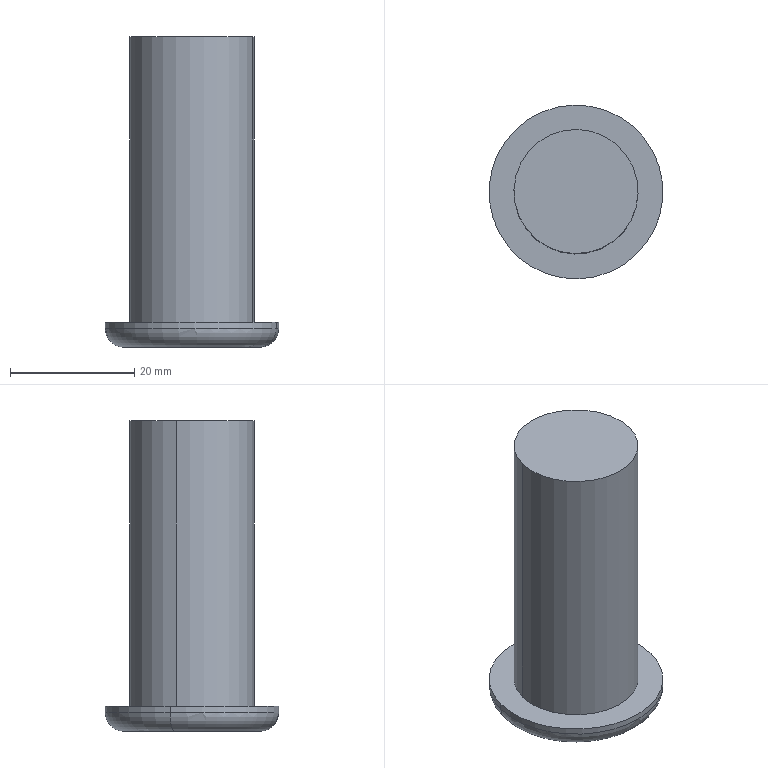Component | SolidWorks | FixedMainPin42mm-1 | 1 solid | 9 faces | box 28 x 28 x 50 mm | volume 16753 mm3 | cylinder 4 | plane 3 | torus 2 | commonest cylinder face diameters 28 x2 20 x2
build123d program:
from build123d import *

# Parameters (mm, degrees)
SKETCH1_R           = 10
BOSS_EXTRUDE1_DEPTH = 42
SKETCH2_R           = 10
BOSS_EXTRUDE2_DEPTH = 4
SKETCH3_R           = 14
BOSS_EXTRUDE3_DEPTH = 4
FILLET2_R           = 3


with BuildPart() as part:
    # Sketch1 → Boss-Extrude1 (new body)
    with BuildSketch(Plane.XY):
        with Locations(Location((0, 0, 0), (0, 0, 180))):
            Circle(SKETCH1_R)
    extrude(amount=BOSS_EXTRUDE1_DEPTH)

    # Sketch2 → Boss-Extrude2 (add)
    with BuildSketch(Plane.XY.offset(42)):
        with Locations(Location((0, 0, 0), (0, 0, 180))):
            Circle(SKETCH2_R)
    extrude(amount=BOSS_EXTRUDE2_DEPTH)

    # Sketch3 → Boss-Extrude3 (add)
    with BuildSketch(Plane.XY.offset(46)):
        Circle(SKETCH3_R)
    extrude(amount=BOSS_EXTRUDE3_DEPTH)

    # Fillet2
    fillet2_edges = [part.edges().sort_by_distance(p)[0] for p in [
        (-14, 0, 50),
    ]]
    fillet(fillet2_edges, radius=FILLET2_R)


solid = part.part

# Placed as in the assembly
solid = solid.moved(Location((17.47, 39.391, 160.846), (180, 0, 0)))
STEP:
#1=CARTESIAN_POINT('',(1.221,1.411,4.482));
#2=VERTEX_POINT('',#1);
#3=CARTESIAN_POINT('',(0.1545,1.69,4.482));
#4=VERTEX_POINT('',#3);
#5=CARTESIAN_POINT('',(0.6878,1.551,4.482));
#6=DIRECTION('',(0.,0.,1.));
#7=DIRECTION('',(-0.9675,0.2528,0.));
#8=AXIS2_PLACEMENT_3D('',#5,#6,#7);
#9=CIRCLE('',#8,0.5512);
#10=EDGE_CURVE('',#2,#4,#9,.T.);
#11=ORIENTED_EDGE('',*,*,#10,.F.);
#12=CARTESIAN_POINT('',(1.107,1.441,4.364));
#13=VERTEX_POINT('',#12);
#14=CARTESIAN_POINT('',(1.107,1.441,4.482));
#15=DIRECTION('',(0.2528,0.9675,0.));
#16=DIRECTION('',(-0.9675,0.2528,0.));
#17=AXIS2_PLACEMENT_3D('',#14,#15,#16);
#18=CIRCLE('',#17,0.1181);
#19=EDGE_CURVE('',#2,#13,#18,.T.);
#20=ORIENTED_EDGE('',*,*,#19,.T.);
#21=CARTESIAN_POINT('',(0.2688,1.66,4.364));
#22=VERTEX_POINT('',#21);
#23=CARTESIAN_POINT('',(0.6878,1.551,4.364));
#24=DIRECTION('',(0.,0.,-1.));
#25=DIRECTION('',(-0.9675,0.2528,0.));
#26=AXIS2_PLACEMENT_3D('',#23,#24,#25);
#27=CIRCLE('',#26,0.4331);
#28=EDGE_CURVE('',#22,#13,#27,.T.);
#29=ORIENTED_EDGE('',*,*,#28,.F.);
#30=CARTESIAN_POINT('',(0.2688,1.66,4.482));
#31=DIRECTION('',(-0.2528,-0.9675,0.));
#32=DIRECTION('',(0.9675,-0.2528,0.));
#33=AXIS2_PLACEMENT_3D('',#30,#31,#32);
#34=CIRCLE('',#33,0.1181);
#35=EDGE_CURVE('',#4,#22,#34,.T.);
#36=ORIENTED_EDGE('',*,*,#35,.F.);
#37=EDGE_LOOP('',(#11,#20,#29,#36));
#38=FACE_OUTER_BOUND('',#37,.T.);
#39=CARTESIAN_POINT('',(0.6878,1.551,4.482));
#40=DIRECTION('',(0.,0.,-1.));
#41=DIRECTION('',(-0.9675,0.2528,0.));
#42=AXIS2_PLACEMENT_3D('',#39,#40,#41);
#43=TOROIDAL_SURFACE('',#42,0.4331,0.1181);
#44=ADVANCED_FACE('',(#38),#43,.T.);
#45=ORIENTED_EDGE('',*,*,#10,.T.);
#46=CARTESIAN_POINT('',(0.1545,1.69,4.521));
#47=VERTEX_POINT('',#46);
#48=CARTESIAN_POINT('',(0.1545,1.69,4.364));
#49=DIRECTION('',(0.,0.,1.));
#50=VECTOR('',#49,39.37);
#51=LINE('',#48,#50);
#52=EDGE_CURVE('',#4,#47,#51,.T.);
#53=ORIENTED_EDGE('',*,*,#52,.T.);
#54=CARTESIAN_POINT('',(1.221,1.411,4.521));
#55=VERTEX_POINT('',#54);
#56=CARTESIAN_POINT('',(0.6878,1.551,4.521));
#57=DIRECTION('',(0.,0.,-1.));
#58=DIRECTION('',(-0.9675,0.2528,0.));
#59=AXIS2_PLACEMENT_3D('',#56,#57,#58);
#60=CIRCLE('',#59,0.5512);
#61=EDGE_CURVE('',#47,#55,#60,.T.);
#62=ORIENTED_EDGE('',*,*,#61,.T.);
#63=CARTESIAN_POINT('',(1.221,1.411,4.364));
#64=DIRECTION('',(0.,0.,1.));
#65=VECTOR('',#64,39.37);
#66=LINE('',#63,#65);
#67=EDGE_CURVE('',#2,#55,#66,.T.);
#68=ORIENTED_EDGE('',*,*,#67,.F.);
#69=EDGE_LOOP('',(#45,#53,#62,#68));
#70=FACE_OUTER_BOUND('',#69,.T.);
#71=CARTESIAN_POINT('',(0.6878,1.551,4.364));
#72=DIRECTION('',(0.,0.,1.));
#73=DIRECTION('',(0.9675,-0.2528,0.));
#74=AXIS2_PLACEMENT_3D('',#71,#72,#73);
#75=CYLINDRICAL_SURFACE('',#74,0.5512);
#76=ADVANCED_FACE('',(#70),#75,.T.);
#77=CARTESIAN_POINT('',(0.3069,1.65,4.521));
#78=VERTEX_POINT('',#77);
#79=CARTESIAN_POINT('',(1.069,1.451,4.521));
#80=VERTEX_POINT('',#79);
#81=CARTESIAN_POINT('',(0.6878,1.551,4.521));
#82=DIRECTION('',(0.,0.,-1.));
#83=DIRECTION('',(-0.9675,0.2528,0.));
#84=AXIS2_PLACEMENT_3D('',#81,#82,#83);
#85=CIRCLE('',#84,0.3937);
#86=EDGE_CURVE('',#78,#80,#85,.T.);
#87=ORIENTED_EDGE('',*,*,#86,.F.);
#88=CARTESIAN_POINT('',(0.3069,1.65,6.333));
#89=VERTEX_POINT('',#88);
#90=CARTESIAN_POINT('',(0.3069,1.65,4.679));
#91=DIRECTION('',(0.,0.,1.));
#92=VECTOR('',#91,39.37);
#93=LINE('',#90,#92);
#94=EDGE_CURVE('',#78,#89,#93,.T.);
#95=ORIENTED_EDGE('',*,*,#94,.T.);
#96=CARTESIAN_POINT('',(1.069,1.451,6.333));
#97=VERTEX_POINT('',#96);
#98=CARTESIAN_POINT('',(0.6878,1.551,6.333));
#99=DIRECTION('',(0.,0.,-1.));
#100=DIRECTION('',(-0.9675,0.2528,0.));
#101=AXIS2_PLACEMENT_3D('',#98,#99,#100);
#102=CIRCLE('',#101,0.3937);
#103=EDGE_CURVE('',#89,#97,#102,.T.);
#104=ORIENTED_EDGE('',*,*,#103,.T.);
#105=CARTESIAN_POINT('',(1.069,1.451,4.679));
#106=DIRECTION('',(0.,0.,1.));
#107=VECTOR('',#106,39.37);
#108=LINE('',#105,#107);
#109=EDGE_CURVE('',#80,#97,#108,.T.);
#110=ORIENTED_EDGE('',*,*,#109,.F.);
#111=EDGE_LOOP('',(#87,#95,#104,#110));
#112=FACE_OUTER_BOUND('',#111,.T.);
#113=CARTESIAN_POINT('',(0.6878,1.551,4.679));
#114=DIRECTION('',(0.,0.,1.));
#115=DIRECTION('',(0.9675,-0.2528,0.));
#116=AXIS2_PLACEMENT_3D('',#113,#114,#115);
#117=CYLINDRICAL_SURFACE('',#116,0.3937);
#118=ADVANCED_FACE('',(#112),#117,.T.);
#119=ORIENTED_EDGE('',*,*,#94,.F.);
#120=CARTESIAN_POINT('',(0.6878,1.551,4.521));
#121=DIRECTION('',(0.,0.,-1.));
#122=DIRECTION('',(-0.9675,0.2528,0.));
#123=AXIS2_PLACEMENT_3D('',#120,#121,#122);
#124=CIRCLE('',#123,0.3937);
#125=EDGE_CURVE('',#80,#78,#124,.T.);
#126=ORIENTED_EDGE('',*,*,#125,.F.);
#127=ORIENTED_EDGE('',*,*,#109,.T.);
#128=CARTESIAN_POINT('',(0.6878,1.551,6.333));
#129=DIRECTION('',(0.,0.,-1.));
#130=DIRECTION('',(-0.9675,0.2528,0.));
#131=AXIS2_PLACEMENT_3D('',#128,#129,#130);
#132=CIRCLE('',#131,0.3937);
#133=EDGE_CURVE('',#97,#89,#132,.T.);
#134=ORIENTED_EDGE('',*,*,#133,.T.);
#135=EDGE_LOOP('',(#119,#126,#127,#134));
#136=FACE_OUTER_BOUND('',#135,.T.);
#137=CARTESIAN_POINT('',(0.6878,1.551,4.679));
#138=DIRECTION('',(0.,0.,1.));
#139=DIRECTION('',(0.9675,-0.2528,0.));
#140=AXIS2_PLACEMENT_3D('',#137,#138,#139);
#141=CYLINDRICAL_SURFACE('',#140,0.3937);
#142=ADVANCED_FACE('',(#136),#141,.T.);
#143=ORIENTED_EDGE('',*,*,#133,.F.);
#144=ORIENTED_EDGE('',*,*,#103,.F.);
#145=EDGE_LOOP('',(#143,#144));
#146=FACE_OUTER_BOUND('',#145,.T.);
#147=CARTESIAN_POINT('',(0.6878,1.551,6.333));
#148=DIRECTION('',(0.,0.,-1.));
#149=DIRECTION('',(-0.9675,0.2528,0.));
#150=AXIS2_PLACEMENT_3D('',#147,#148,#149);
#151=PLANE('',#150);
#152=ADVANCED_FACE('',(#146),#151,.F.);
#153=ORIENTED_EDGE('',*,*,#52,.F.);
#154=CARTESIAN_POINT('',(0.6878,1.551,4.482));
#155=DIRECTION('',(0.,0.,1.));
#156=DIRECTION('',(-0.9675,0.2528,0.));
#157=AXIS2_PLACEMENT_3D('',#154,#155,#156);
#158=CIRCLE('',#157,0.5512);
#159=EDGE_CURVE('',#4,#2,#158,.T.);
#160=ORIENTED_EDGE('',*,*,#159,.T.);
#161=ORIENTED_EDGE('',*,*,#67,.T.);
#162=CARTESIAN_POINT('',(0.6878,1.551,4.521));
#163=DIRECTION('',(0.,0.,-1.));
#164=DIRECTION('',(-0.9675,0.2528,0.));
#165=AXIS2_PLACEMENT_3D('',#162,#163,#164);
#166=CIRCLE('',#165,0.5512);
#167=EDGE_CURVE('',#55,#47,#166,.T.);
#168=ORIENTED_EDGE('',*,*,#167,.T.);
#169=EDGE_LOOP('',(#153,#160,#161,#168));
#170=FACE_OUTER_BOUND('',#169,.T.);
#171=CARTESIAN_POINT('',(0.6878,1.551,4.364));
#172=DIRECTION('',(0.,0.,1.));
#173=DIRECTION('',(0.9675,-0.2528,0.));
#174=AXIS2_PLACEMENT_3D('',#171,#172,#173);
#175=CYLINDRICAL_SURFACE('',#174,0.5512);
#176=ADVANCED_FACE('',(#170),#175,.T.);
#177=ORIENTED_EDGE('',*,*,#28,.T.);
#178=CARTESIAN_POINT('',(0.6878,1.551,4.364));
#179=DIRECTION('',(0.,0.,-1.));
#180=DIRECTION('',(-0.9675,0.2528,0.));
#181=AXIS2_PLACEMENT_3D('',#178,#179,#180);
#182=CIRCLE('',#181,0.4331);
#183=EDGE_CURVE('',#13,#22,#182,.T.);
#184=ORIENTED_EDGE('',*,*,#183,.T.);
#185=EDGE_LOOP('',(#177,#184));
#186=FACE_OUTER_BOUND('',#185,.T.);
#187=CARTESIAN_POINT('',(0.6878,1.551,4.364));
#188=DIRECTION('',(0.,0.,-1.));
#189=DIRECTION('',(-0.9675,0.2528,0.));
#190=AXIS2_PLACEMENT_3D('',#187,#188,#189);
#191=PLANE('',#190);
#192=ADVANCED_FACE('',(#186),#191,.T.);
#193=ORIENTED_EDGE('',*,*,#125,.T.);
#194=ORIENTED_EDGE('',*,*,#86,.T.);
#195=EDGE_LOOP('',(#193,#194));
#196=FACE_BOUND('',#195,.T.);
#197=ORIENTED_EDGE('',*,*,#167,.F.);
#198=ORIENTED_EDGE('',*,*,#61,.F.);
#199=EDGE_LOOP('',(#197,#198));
#200=FACE_OUTER_BOUND('',#199,.T.);
#201=CARTESIAN_POINT('',(0.6878,1.551,4.521));
#202=DIRECTION('',(0.,0.,-1.));
#203=DIRECTION('',(-0.9675,0.2528,0.));
#204=AXIS2_PLACEMENT_3D('',#201,#202,#203);
#205=PLANE('',#204);
#206=ADVANCED_FACE('',(#196,#200),#205,.F.);
#207=ORIENTED_EDGE('',*,*,#19,.F.);
#208=ORIENTED_EDGE('',*,*,#159,.F.);
#209=ORIENTED_EDGE('',*,*,#35,.T.);
#210=ORIENTED_EDGE('',*,*,#183,.F.);
#211=EDGE_LOOP('',(#207,#208,#209,#210));
#212=FACE_OUTER_BOUND('',#211,.T.);
#213=CARTESIAN_POINT('',(0.6878,1.551,4.482));
#214=DIRECTION('',(0.,0.,-1.));
#215=DIRECTION('',(-0.9675,0.2528,0.));
#216=AXIS2_PLACEMENT_3D('',#213,#214,#215);
#217=TOROIDAL_SURFACE('',#216,0.4331,0.1181);
#218=ADVANCED_FACE('',(#212),#217,.T.);
#219=CLOSED_SHELL('',(#44,#76,#118,#142,#152,#176,#192,#206,#218));
#220=MANIFOLD_SOLID_BREP('',#219);
#221=CARTESIAN_POINT('',(0.,0.,0.));
#222=DIRECTION('',(0.,0.,1.));
#223=DIRECTION('',(1.,0.,0.));
#224=AXIS2_PLACEMENT_3D('',#221,#222,#223);
#225=(LENGTH_UNIT()NAMED_UNIT(*)SI_UNIT($,.METRE.));
#226=LENGTH_MEASURE_WITH_UNIT(LENGTH_MEASURE(0.0254),#225);
#227=DIMENSIONAL_EXPONENTS(1.,0.,0.,0.,0.,0.,0.);
#228=(CONVERSION_BASED_UNIT('',#226)LENGTH_UNIT()NAMED_UNIT(#227));
#229=UNCERTAINTY_MEASURE_WITH_UNIT(LENGTH_MEASURE(0.00001),#228,'','');
#230=(NAMED_UNIT(*)PLANE_ANGLE_UNIT()SI_UNIT($,.RADIAN.));
#231=(NAMED_UNIT(*)SI_UNIT($,.STERADIAN.)SOLID_ANGLE_UNIT());
#232=(GEOMETRIC_REPRESENTATION_CONTEXT(3)GLOBAL_UNCERTAINTY_ASSIGNED_CONTEXT((#229))GLOBAL_UNIT_ASSIGNED_CONTEXT((#228,#230,#231))REPRESENTATION_CONTEXT('',''));
#233=ADVANCED_BREP_SHAPE_REPRESENTATION('',(#220,#224),#232);
#234=COLOUR_RGB('',0.7922,0.8196,0.9333);
#235=FILL_AREA_STYLE_COLOUR('',#234);
#236=FILL_AREA_STYLE('',(#235));
#237=SURFACE_STYLE_FILL_AREA(#236);
#238=SURFACE_SIDE_STYLE('',(#237));
#239=SURFACE_STYLE_USAGE(.BOTH.,#238);
#240=PRESENTATION_STYLE_ASSIGNMENT((#239));
#241=STYLED_ITEM('',(#240),#220);
#242=PRESENTATION_LAYER_ASSIGNMENT('','',(#241));
#243=(LENGTH_UNIT()NAMED_UNIT(*)SI_UNIT($,.METRE.));
#244=LENGTH_MEASURE_WITH_UNIT(LENGTH_MEASURE(0.0254),#243);
#245=DIMENSIONAL_EXPONENTS(1.,0.,0.,0.,0.,0.,0.);
#246=(CONVERSION_BASED_UNIT('',#244)LENGTH_UNIT()NAMED_UNIT(#245));
#247=UNCERTAINTY_MEASURE_WITH_UNIT(LENGTH_MEASURE(0.00001),#246,'','');
#248=(NAMED_UNIT(*)PLANE_ANGLE_UNIT()SI_UNIT($,.RADIAN.));
#249=(NAMED_UNIT(*)SI_UNIT($,.STERADIAN.)SOLID_ANGLE_UNIT());
#250=(GEOMETRIC_REPRESENTATION_CONTEXT(3)GLOBAL_UNCERTAINTY_ASSIGNED_CONTEXT((#247))GLOBAL_UNIT_ASSIGNED_CONTEXT((#246,#248,#249))REPRESENTATION_CONTEXT('',''));
#251=MECHANICAL_DESIGN_GEOMETRIC_PRESENTATION_REPRESENTATION('',(#241),#250);